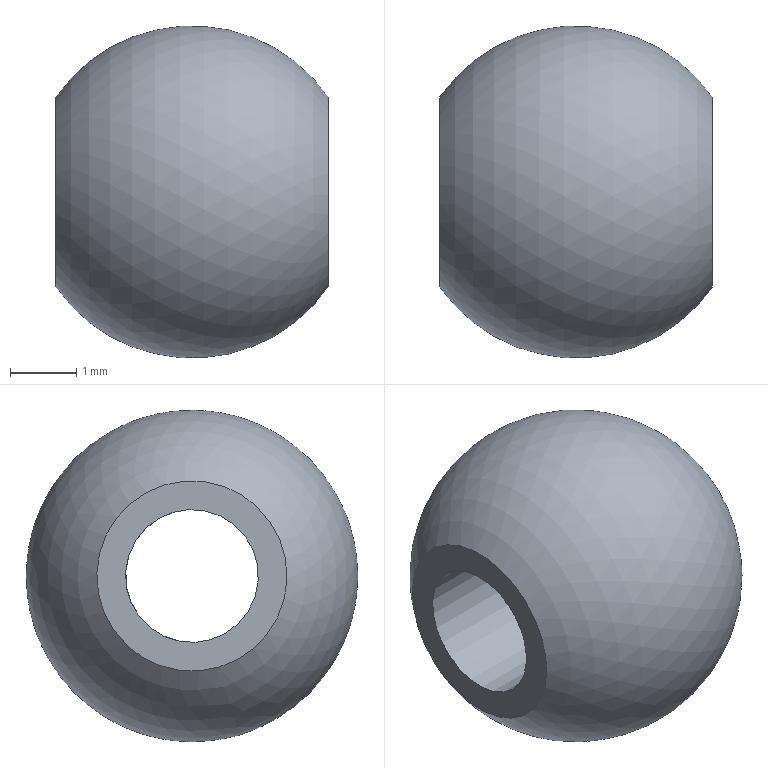Component | NX | BALL_1_2 | 1 solid | 4 faces | box 4.1 x 5 x 5 mm | volume 50 mm3 | plane 2 | sphere 1 | cylinder 1 | commonest cylinder face diameters 2 x1
STEP:
#1=CARTESIAN_POINT('',(0.,0.,0.));
#2=DIRECTION('',(0.,0.,1.));
#3=DIRECTION('',(1.,0.,0.));
#4=AXIS2_PLACEMENT_3D('',#1,#2,#3);
#5=CARTESIAN_POINT('',(49.212,-56.394,49.81));
#6=VERTEX_POINT('',#5);
#7=CARTESIAN_POINT('',(49.212,-55.987,51.182));
#8=DIRECTION('',(-1.,0.0007539,-0.00000421));
#9=DIRECTION('',(-0.00021,-0.2839,-0.9588));
#10=AXIS2_PLACEMENT_3D('',#7,#8,#9);
#11=CIRCLE('',#10,1.431);
#12=CARTESIAN_POINT('',(47.162,-55.986,51.182));
#13=DIRECTION('',(1.,-0.0007539,0.00000421));
#14=DIRECTION('',(-0.00021,-0.2839,-0.9588));
#15=AXIS2_PLACEMENT_3D('',#12,#13,#14);
#16=SPHERICAL_SURFACE('',#15,2.5);
#17=CARTESIAN_POINT('',(6.283,0.9614));
#18=CARTESIAN_POINT('',(6.188,0.9614));
#19=CARTESIAN_POINT('',(5.998,0.9614));
#20=CARTESIAN_POINT('',(5.712,0.9614));
#21=CARTESIAN_POINT('',(5.426,0.9614));
#22=CARTESIAN_POINT('',(5.141,0.9614));
#23=CARTESIAN_POINT('',(4.855,0.9614));
#24=CARTESIAN_POINT('',(4.57,0.9614));
#25=CARTESIAN_POINT('',(4.284,0.9614));
#26=CARTESIAN_POINT('',(3.998,0.9614));
#27=CARTESIAN_POINT('',(3.713,0.9614));
#28=CARTESIAN_POINT('',(3.427,0.9614));
#29=CARTESIAN_POINT('',(3.142,0.9614));
#30=CARTESIAN_POINT('',(2.856,0.9614));
#31=CARTESIAN_POINT('',(2.57,0.9614));
#32=CARTESIAN_POINT('',(2.285,0.9614));
#33=CARTESIAN_POINT('',(1.999,0.9614));
#34=CARTESIAN_POINT('',(1.714,0.9614));
#35=CARTESIAN_POINT('',(1.428,0.9614));
#36=CARTESIAN_POINT('',(1.142,0.9614));
#37=CARTESIAN_POINT('',(0.8568,0.9614));
#38=CARTESIAN_POINT('',(0.5712,0.9614));
#39=CARTESIAN_POINT('',(0.2856,0.9614));
#40=CARTESIAN_POINT('',(0.0952,0.9614));
#41=CARTESIAN_POINT('',(-0.,0.9614));
#42=B_SPLINE_CURVE_WITH_KNOTS('',3,(#17,#18,#19,#20,#21,#22,#23,#24,#25,#26,#27,#28,#29,#30,#31,#32,#33,#34,#35,#36,#37,#38,#39,#40,#41),.UNSPECIFIED.,.F.,.F.,(4,1,1,1,1,1,1,1,1,1,1,1,1,1,1,1,1,1,1,1,1,1,4),(0.,0.2856,0.5712,0.8568,1.142,1.428,1.714,1.999,2.285,2.57,2.856,3.142,3.427,3.713,3.998,4.284,4.57,4.855,5.141,5.426,5.712,5.998,6.283),.QUASI_UNIFORM_KNOTS.);
#43=(GEOMETRIC_REPRESENTATION_CONTEXT(2)PARAMETRIC_REPRESENTATION_CONTEXT()REPRESENTATION_CONTEXT('',''));
#44=DEFINITIONAL_REPRESENTATION('',(#42),#43);
#45=PCURVE('',#16,#44);
#46=CARTESIAN_POINT('',(49.212,-55.987,51.182));
#47=DIRECTION('',(1.,-0.0007539,0.00000421));
#48=DIRECTION('',(-0.00021,-0.2839,-0.9588));
#49=AXIS2_PLACEMENT_3D('',#46,#47,#48);
#50=PLANE('',#49);
#51=CARTESIAN_POINT('',(1.431,0.));
#52=CARTESIAN_POINT('',(1.431,-2.478));
#53=CARTESIAN_POINT('',(-0.7155,-1.239));
#54=CARTESIAN_POINT('',(-2.862,-0.));
#55=CARTESIAN_POINT('',(-0.7155,1.239));
#56=CARTESIAN_POINT('',(1.431,2.478));
#57=CARTESIAN_POINT('',(1.431,0.));
#58=(BOUNDED_CURVE()B_SPLINE_CURVE(2,(#51,#52,#53,#54,#55,#56,#57),.UNSPECIFIED.,.T.,.F.)B_SPLINE_CURVE_WITH_KNOTS((1,2,2,2,2,1),(-2.094,0.,2.094,4.189,6.283,8.378),.UNSPECIFIED.)CURVE()GEOMETRIC_REPRESENTATION_ITEM()RATIONAL_B_SPLINE_CURVE((1.,0.5,1.,0.5,1.,0.5,1.))REPRESENTATION_ITEM(''));
#59=(GEOMETRIC_REPRESENTATION_CONTEXT(2)PARAMETRIC_REPRESENTATION_CONTEXT()REPRESENTATION_CONTEXT('',''));
#60=DEFINITIONAL_REPRESENTATION('',(#58),#59);
#61=PCURVE('',#50,#60);
#62=SURFACE_CURVE('',#11,(#45,#61),.PCURVE_S1.);
#63=EDGE_CURVE('',#6,#6,#62,.T.);
#64=ORIENTED_EDGE('',*,*,#63,.T.);
#65=CARTESIAN_POINT('',(45.112,-56.391,49.81));
#66=VERTEX_POINT('',#65);
#67=CARTESIAN_POINT('',(45.112,-56.391,49.81));
#68=CARTESIAN_POINT('',(45.505,-56.551,49.27));
#69=CARTESIAN_POINT('',(46.078,-56.675,48.851));
#70=CARTESIAN_POINT('',(46.784,-56.745,48.619));
#71=CARTESIAN_POINT('',(47.539,-56.745,48.619));
#72=CARTESIAN_POINT('',(48.245,-56.677,48.851));
#73=CARTESIAN_POINT('',(48.819,-56.553,49.27));
#74=CARTESIAN_POINT('',(49.212,-56.394,49.81));
#75=B_SPLINE_CURVE_WITH_KNOTS('',7,(#67,#68,#69,#70,#71,#72,#73,#74),.UNSPECIFIED.,.F.,.F.,(8,8),(-0.9614,0.9614),.PIECEWISE_BEZIER_KNOTS.);
#76=CARTESIAN_POINT('',(-0.,0.));
#77=DIRECTION('',(0.,1.));
#78=VECTOR('',#77,1.);
#79=LINE('',#76,#78);
#80=(GEOMETRIC_REPRESENTATION_CONTEXT(2)PARAMETRIC_REPRESENTATION_CONTEXT()REPRESENTATION_CONTEXT('',''));
#81=DEFINITIONAL_REPRESENTATION('',(#79),#80);
#82=PCURVE('',#16,#81);
#83=CARTESIAN_POINT('',(6.283,0.));
#84=DIRECTION('',(0.,1.));
#85=VECTOR('',#84,1.);
#86=LINE('',#83,#85);
#87=(GEOMETRIC_REPRESENTATION_CONTEXT(2)PARAMETRIC_REPRESENTATION_CONTEXT()REPRESENTATION_CONTEXT('',''));
#88=DEFINITIONAL_REPRESENTATION('',(#86),#87);
#89=PCURVE('',#16,#88);
#90=SEAM_CURVE('',#75,(#82,#89),.PCURVE_S1.);
#91=EDGE_CURVE('',#66,#6,#90,.T.);
#92=ORIENTED_EDGE('',*,*,#91,.F.);
#93=CARTESIAN_POINT('',(45.112,-55.578,52.554));
#94=VERTEX_POINT('',#93);
#95=CARTESIAN_POINT('',(45.112,-55.984,51.182));
#96=DIRECTION('',(1.,-0.0007539,0.00000421));
#97=DIRECTION('',(0.00021,0.2839,0.9588));
#98=AXIS2_PLACEMENT_3D('',#95,#96,#97);
#99=CIRCLE('',#98,1.431);
#100=CARTESIAN_POINT('',(-3.142,-0.9614));
#101=CARTESIAN_POINT('',(-3.046,-0.9614));
#102=CARTESIAN_POINT('',(-2.856,-0.9614));
#103=CARTESIAN_POINT('',(-2.57,-0.9614));
#104=CARTESIAN_POINT('',(-2.285,-0.9614));
#105=CARTESIAN_POINT('',(-1.999,-0.9614));
#106=CARTESIAN_POINT('',(-1.714,-0.9614));
#107=CARTESIAN_POINT('',(-1.428,-0.9614));
#108=CARTESIAN_POINT('',(-1.142,-0.9614));
#109=CARTESIAN_POINT('',(-0.8568,-0.9614));
#110=CARTESIAN_POINT('',(-0.5712,-0.9614));
#111=CARTESIAN_POINT('',(-0.2856,-0.9614));
#112=CARTESIAN_POINT('',(-0.,-0.9614));
#113=CARTESIAN_POINT('',(0.2856,-0.9614));
#114=CARTESIAN_POINT('',(0.5712,-0.9614));
#115=CARTESIAN_POINT('',(0.8568,-0.9614));
#116=CARTESIAN_POINT('',(1.142,-0.9614));
#117=CARTESIAN_POINT('',(1.428,-0.9614));
#118=CARTESIAN_POINT('',(1.714,-0.9614));
#119=CARTESIAN_POINT('',(1.999,-0.9614));
#120=CARTESIAN_POINT('',(2.285,-0.9614));
#121=CARTESIAN_POINT('',(2.57,-0.9614));
#122=CARTESIAN_POINT('',(2.856,-0.9614));
#123=CARTESIAN_POINT('',(3.046,-0.9614));
#124=CARTESIAN_POINT('',(3.142,-0.9614));
#125=B_SPLINE_CURVE_WITH_KNOTS('',3,(#100,#101,#102,#103,#104,#105,#106,#107,#108,#109,#110,#111,#112,#113,#114,#115,#116,#117,#118,#119,#120,#121,#122,#123,#124),.UNSPECIFIED.,.F.,.F.,(4,1,1,1,1,1,1,1,1,1,1,1,1,1,1,1,1,1,1,1,1,1,4),(0.,0.2856,0.5712,0.8568,1.142,1.428,1.714,1.999,2.285,2.57,2.856,3.142,3.427,3.713,3.998,4.284,4.57,4.855,5.141,5.426,5.712,5.998,6.283),.QUASI_UNIFORM_KNOTS.);
#126=(GEOMETRIC_REPRESENTATION_CONTEXT(2)PARAMETRIC_REPRESENTATION_CONTEXT()REPRESENTATION_CONTEXT('',''));
#127=DEFINITIONAL_REPRESENTATION('',(#125),#126);
#128=PCURVE('',#16,#127);
#129=CARTESIAN_POINT('',(45.112,-55.984,51.182));
#130=DIRECTION('',(-1.,0.0007539,-0.00000421));
#131=DIRECTION('',(0.00021,0.2839,0.9588));
#132=AXIS2_PLACEMENT_3D('',#129,#130,#131);
#133=PLANE('',#132);
#134=CARTESIAN_POINT('',(1.431,-0.));
#135=CARTESIAN_POINT('',(1.431,-2.478));
#136=CARTESIAN_POINT('',(-0.7155,-1.239));
#137=CARTESIAN_POINT('',(-2.862,0.));
#138=CARTESIAN_POINT('',(-0.7155,1.239));
#139=CARTESIAN_POINT('',(1.431,2.478));
#140=CARTESIAN_POINT('',(1.431,-0.));
#141=(BOUNDED_CURVE()B_SPLINE_CURVE(2,(#134,#135,#136,#137,#138,#139,#140),.UNSPECIFIED.,.T.,.F.)B_SPLINE_CURVE_WITH_KNOTS((1,2,2,2,2,1),(-2.094,0.,2.094,4.189,6.283,8.378),.UNSPECIFIED.)CURVE()GEOMETRIC_REPRESENTATION_ITEM()RATIONAL_B_SPLINE_CURVE((1.,0.5,1.,0.5,1.,0.5,1.))REPRESENTATION_ITEM(''));
#142=(GEOMETRIC_REPRESENTATION_CONTEXT(2)PARAMETRIC_REPRESENTATION_CONTEXT()REPRESENTATION_CONTEXT('',''));
#143=DEFINITIONAL_REPRESENTATION('',(#141),#142);
#144=PCURVE('',#133,#143);
#145=SURFACE_CURVE('',#99,(#128,#144),.PCURVE_S1.);
#146=EDGE_CURVE('',#66,#94,#145,.T.);
#147=ORIENTED_EDGE('',*,*,#146,.T.);
#148=CARTESIAN_POINT('',(45.112,-55.984,51.182));
#149=DIRECTION('',(1.,-0.0007539,0.00000421));
#150=DIRECTION('',(0.00021,0.2839,0.9588));
#151=AXIS2_PLACEMENT_3D('',#148,#149,#150);
#152=CIRCLE('',#151,1.431);
#153=CARTESIAN_POINT('',(3.142,-0.9614));
#154=CARTESIAN_POINT('',(3.237,-0.9614));
#155=CARTESIAN_POINT('',(3.427,-0.9614));
#156=CARTESIAN_POINT('',(3.713,-0.9614));
#157=CARTESIAN_POINT('',(3.998,-0.9614));
#158=CARTESIAN_POINT('',(4.284,-0.9614));
#159=CARTESIAN_POINT('',(4.57,-0.9614));
#160=CARTESIAN_POINT('',(4.855,-0.9614));
#161=CARTESIAN_POINT('',(5.141,-0.9614));
#162=CARTESIAN_POINT('',(5.426,-0.9614));
#163=CARTESIAN_POINT('',(5.712,-0.9614));
#164=CARTESIAN_POINT('',(5.998,-0.9614));
#165=CARTESIAN_POINT('',(6.283,-0.9614));
#166=CARTESIAN_POINT('',(6.569,-0.9614));
#167=CARTESIAN_POINT('',(6.854,-0.9614));
#168=CARTESIAN_POINT('',(7.14,-0.9614));
#169=CARTESIAN_POINT('',(7.426,-0.9614));
#170=CARTESIAN_POINT('',(7.711,-0.9614));
#171=CARTESIAN_POINT('',(7.997,-0.9614));
#172=CARTESIAN_POINT('',(8.282,-0.9614));
#173=CARTESIAN_POINT('',(8.568,-0.9614));
#174=CARTESIAN_POINT('',(8.854,-0.9614));
#175=CARTESIAN_POINT('',(9.139,-0.9614));
#176=CARTESIAN_POINT('',(9.33,-0.9614));
#177=CARTESIAN_POINT('',(9.425,-0.9614));
#178=B_SPLINE_CURVE_WITH_KNOTS('',3,(#153,#154,#155,#156,#157,#158,#159,#160,#161,#162,#163,#164,#165,#166,#167,#168,#169,#170,#171,#172,#173,#174,#175,#176,#177),.UNSPECIFIED.,.F.,.F.,(4,1,1,1,1,1,1,1,1,1,1,1,1,1,1,1,1,1,1,1,1,1,4),(0.,0.2856,0.5712,0.8568,1.142,1.428,1.714,1.999,2.285,2.57,2.856,3.142,3.427,3.713,3.998,4.284,4.57,4.855,5.141,5.426,5.712,5.998,6.283),.QUASI_UNIFORM_KNOTS.);
#179=(GEOMETRIC_REPRESENTATION_CONTEXT(2)PARAMETRIC_REPRESENTATION_CONTEXT()REPRESENTATION_CONTEXT('',''));
#180=DEFINITIONAL_REPRESENTATION('',(#178),#179);
#181=PCURVE('',#16,#180);
#182=CARTESIAN_POINT('',(1.431,-0.));
#183=CARTESIAN_POINT('',(1.431,-2.478));
#184=CARTESIAN_POINT('',(-0.7155,-1.239));
#185=CARTESIAN_POINT('',(-2.862,0.));
#186=CARTESIAN_POINT('',(-0.7155,1.239));
#187=CARTESIAN_POINT('',(1.431,2.478));
#188=CARTESIAN_POINT('',(1.431,-0.));
#189=(BOUNDED_CURVE()B_SPLINE_CURVE(2,(#182,#183,#184,#185,#186,#187,#188),.UNSPECIFIED.,.T.,.F.)B_SPLINE_CURVE_WITH_KNOTS((1,2,2,2,2,1),(-2.094,0.,2.094,4.189,6.283,8.378),.UNSPECIFIED.)CURVE()GEOMETRIC_REPRESENTATION_ITEM()RATIONAL_B_SPLINE_CURVE((1.,0.5,1.,0.5,1.,0.5,1.))REPRESENTATION_ITEM(''));
#190=(GEOMETRIC_REPRESENTATION_CONTEXT(2)PARAMETRIC_REPRESENTATION_CONTEXT()REPRESENTATION_CONTEXT('',''));
#191=DEFINITIONAL_REPRESENTATION('',(#189),#190);
#192=PCURVE('',#133,#191);
#193=SURFACE_CURVE('',#152,(#181,#192),.PCURVE_S1.);
#194=EDGE_CURVE('',#94,#66,#193,.T.);
#195=ORIENTED_EDGE('',*,*,#194,.T.);
#196=ORIENTED_EDGE('',*,*,#91,.T.);
#197=EDGE_LOOP('',(#64,#92,#147,#195,#196));
#198=FACE_BOUND('',#197,.T.);
#199=ADVANCED_FACE('',(#198),#16,.T.);
#200=CARTESIAN_POINT('',(49.212,-55.703,52.141));
#201=VERTEX_POINT('',#200);
#202=CARTESIAN_POINT('',(49.212,-55.987,51.182));
#203=DIRECTION('',(-1.,0.0007539,-0.00000421));
#204=DIRECTION('',(0.00021,0.2839,0.9588));
#205=AXIS2_PLACEMENT_3D('',#202,#203,#204);
#206=CIRCLE('',#205,1.);
#207=CARTESIAN_POINT('',(-1.,-0.));
#208=CARTESIAN_POINT('',(-1.,1.732));
#209=CARTESIAN_POINT('',(0.5,0.866));
#210=CARTESIAN_POINT('',(2.,0.));
#211=CARTESIAN_POINT('',(0.5,-0.866));
#212=CARTESIAN_POINT('',(-1.,-1.732));
#213=CARTESIAN_POINT('',(-1.,-0.));
#214=(BOUNDED_CURVE()B_SPLINE_CURVE(2,(#207,#208,#209,#210,#211,#212,#213),.UNSPECIFIED.,.T.,.F.)B_SPLINE_CURVE_WITH_KNOTS((1,2,2,2,2,1),(-2.094,0.,2.094,4.189,6.283,8.378),.UNSPECIFIED.)CURVE()GEOMETRIC_REPRESENTATION_ITEM()RATIONAL_B_SPLINE_CURVE((1.,0.5,1.,0.5,1.,0.5,1.))REPRESENTATION_ITEM(''));
#215=(GEOMETRIC_REPRESENTATION_CONTEXT(2)PARAMETRIC_REPRESENTATION_CONTEXT()REPRESENTATION_CONTEXT('',''));
#216=DEFINITIONAL_REPRESENTATION('',(#214),#215);
#217=PCURVE('',#50,#216);
#218=CARTESIAN_POINT('',(49.212,-55.987,51.182));
#219=DIRECTION('',(-1.,0.0007539,-0.00000421));
#220=DIRECTION('',(0.00021,0.2839,0.9588));
#221=AXIS2_PLACEMENT_3D('',#218,#219,#220);
#222=CYLINDRICAL_SURFACE('',#221,1.);
#223=CARTESIAN_POINT('',(0.,0.));
#224=DIRECTION('',(1.,0.));
#225=VECTOR('',#224,1.);
#226=LINE('',#223,#225);
#227=(GEOMETRIC_REPRESENTATION_CONTEXT(2)PARAMETRIC_REPRESENTATION_CONTEXT()REPRESENTATION_CONTEXT('',''));
#228=DEFINITIONAL_REPRESENTATION('',(#226),#227);
#229=PCURVE('',#222,#228);
#230=SURFACE_CURVE('',#206,(#217,#229),.PCURVE_S1.);
#231=EDGE_CURVE('',#201,#201,#230,.T.);
#232=ORIENTED_EDGE('',*,*,#231,.T.);
#233=EDGE_LOOP('',(#232));
#234=FACE_BOUND('',#233,.T.);
#235=ORIENTED_EDGE('',*,*,#63,.F.);
#236=EDGE_LOOP('',(#235));
#237=FACE_BOUND('',#236,.T.);
#238=ADVANCED_FACE('',(#234,#237),#50,.T.);
#239=CARTESIAN_POINT('',(45.112,-55.7,52.141));
#240=VERTEX_POINT('',#239);
#241=CARTESIAN_POINT('',(45.112,-55.984,51.182));
#242=DIRECTION('',(-1.,0.0007539,-0.00000421));
#243=DIRECTION('',(0.00021,0.2839,0.9588));
#244=AXIS2_PLACEMENT_3D('',#241,#242,#243);
#245=CIRCLE('',#244,1.);
#246=CARTESIAN_POINT('',(0.,0.));
#247=DIRECTION('',(1.,-0.));
#248=AXIS2_PLACEMENT_2D('',#246,#247);
#249=CIRCLE('',#248,1.);
#250=(GEOMETRIC_REPRESENTATION_CONTEXT(2)PARAMETRIC_REPRESENTATION_CONTEXT()REPRESENTATION_CONTEXT('',''));
#251=DEFINITIONAL_REPRESENTATION('',(#249),#250);
#252=PCURVE('',#133,#251);
#253=CARTESIAN_POINT('',(0.,4.1));
#254=DIRECTION('',(1.,0.));
#255=VECTOR('',#254,1.);
#256=LINE('',#253,#255);
#257=(GEOMETRIC_REPRESENTATION_CONTEXT(2)PARAMETRIC_REPRESENTATION_CONTEXT()REPRESENTATION_CONTEXT('',''));
#258=DEFINITIONAL_REPRESENTATION('',(#256),#257);
#259=PCURVE('',#222,#258);
#260=SURFACE_CURVE('',#245,(#252,#259),.PCURVE_S1.);
#261=EDGE_CURVE('',#240,#240,#260,.T.);
#262=ORIENTED_EDGE('',*,*,#261,.F.);
#263=EDGE_LOOP('',(#262));
#264=FACE_BOUND('',#263,.T.);
#265=ORIENTED_EDGE('',*,*,#194,.F.);
#266=ORIENTED_EDGE('',*,*,#146,.F.);
#267=EDGE_LOOP('',(#265,#266));
#268=FACE_BOUND('',#267,.T.);
#269=ADVANCED_FACE('',(#264,#268),#133,.T.);
#270=ORIENTED_EDGE('',*,*,#261,.F.);
#271=CARTESIAN_POINT('',(49.212,-55.703,52.141));
#272=CARTESIAN_POINT('',(45.112,-55.7,52.141));
#273=B_SPLINE_CURVE_WITH_KNOTS('',1,(#271,#272),.UNSPECIFIED.,.F.,.F.,(2,2),(0.,4.1),.PIECEWISE_BEZIER_KNOTS.);
#274=CARTESIAN_POINT('',(0.,0.));
#275=DIRECTION('',(0.,1.));
#276=VECTOR('',#275,1.);
#277=LINE('',#274,#276);
#278=(GEOMETRIC_REPRESENTATION_CONTEXT(2)PARAMETRIC_REPRESENTATION_CONTEXT()REPRESENTATION_CONTEXT('',''));
#279=DEFINITIONAL_REPRESENTATION('',(#277),#278);
#280=PCURVE('',#222,#279);
#281=CARTESIAN_POINT('',(6.283,0.));
#282=DIRECTION('',(0.,1.));
#283=VECTOR('',#282,1.);
#284=LINE('',#281,#283);
#285=(GEOMETRIC_REPRESENTATION_CONTEXT(2)PARAMETRIC_REPRESENTATION_CONTEXT()REPRESENTATION_CONTEXT('',''));
#286=DEFINITIONAL_REPRESENTATION('',(#284),#285);
#287=PCURVE('',#222,#286);
#288=SEAM_CURVE('',#273,(#280,#287),.PCURVE_S1.);
#289=EDGE_CURVE('',#201,#240,#288,.T.);
#290=ORIENTED_EDGE('',*,*,#289,.F.);
#291=ORIENTED_EDGE('',*,*,#231,.T.);
#292=ORIENTED_EDGE('',*,*,#289,.T.);
#293=EDGE_LOOP('',(#270,#290,#291,#292));
#294=FACE_BOUND('',#293,.F.);
#295=ADVANCED_FACE('',(#294),#222,.F.);
#296=CLOSED_SHELL('',(#199,#238,#269,#295));
#297=MANIFOLD_SOLID_BREP('',#296);
#298=(LENGTH_UNIT()NAMED_UNIT(*)SI_UNIT(.MILLI.,.METRE.));
#299=UNCERTAINTY_MEASURE_WITH_UNIT(LENGTH_MEASURE(0.000005),#298,'','');
#300=(NAMED_UNIT(*)PLANE_ANGLE_UNIT()SI_UNIT($,.RADIAN.));
#301=(NAMED_UNIT(*)SI_UNIT($,.STERADIAN.)SOLID_ANGLE_UNIT());
#302=(GEOMETRIC_REPRESENTATION_CONTEXT(3)GLOBAL_UNCERTAINTY_ASSIGNED_CONTEXT((#299))GLOBAL_UNIT_ASSIGNED_CONTEXT((#298,#300,#301))REPRESENTATION_CONTEXT('',''));
#303=ADVANCED_BREP_SHAPE_REPRESENTATION('',(#4,#297),#302);